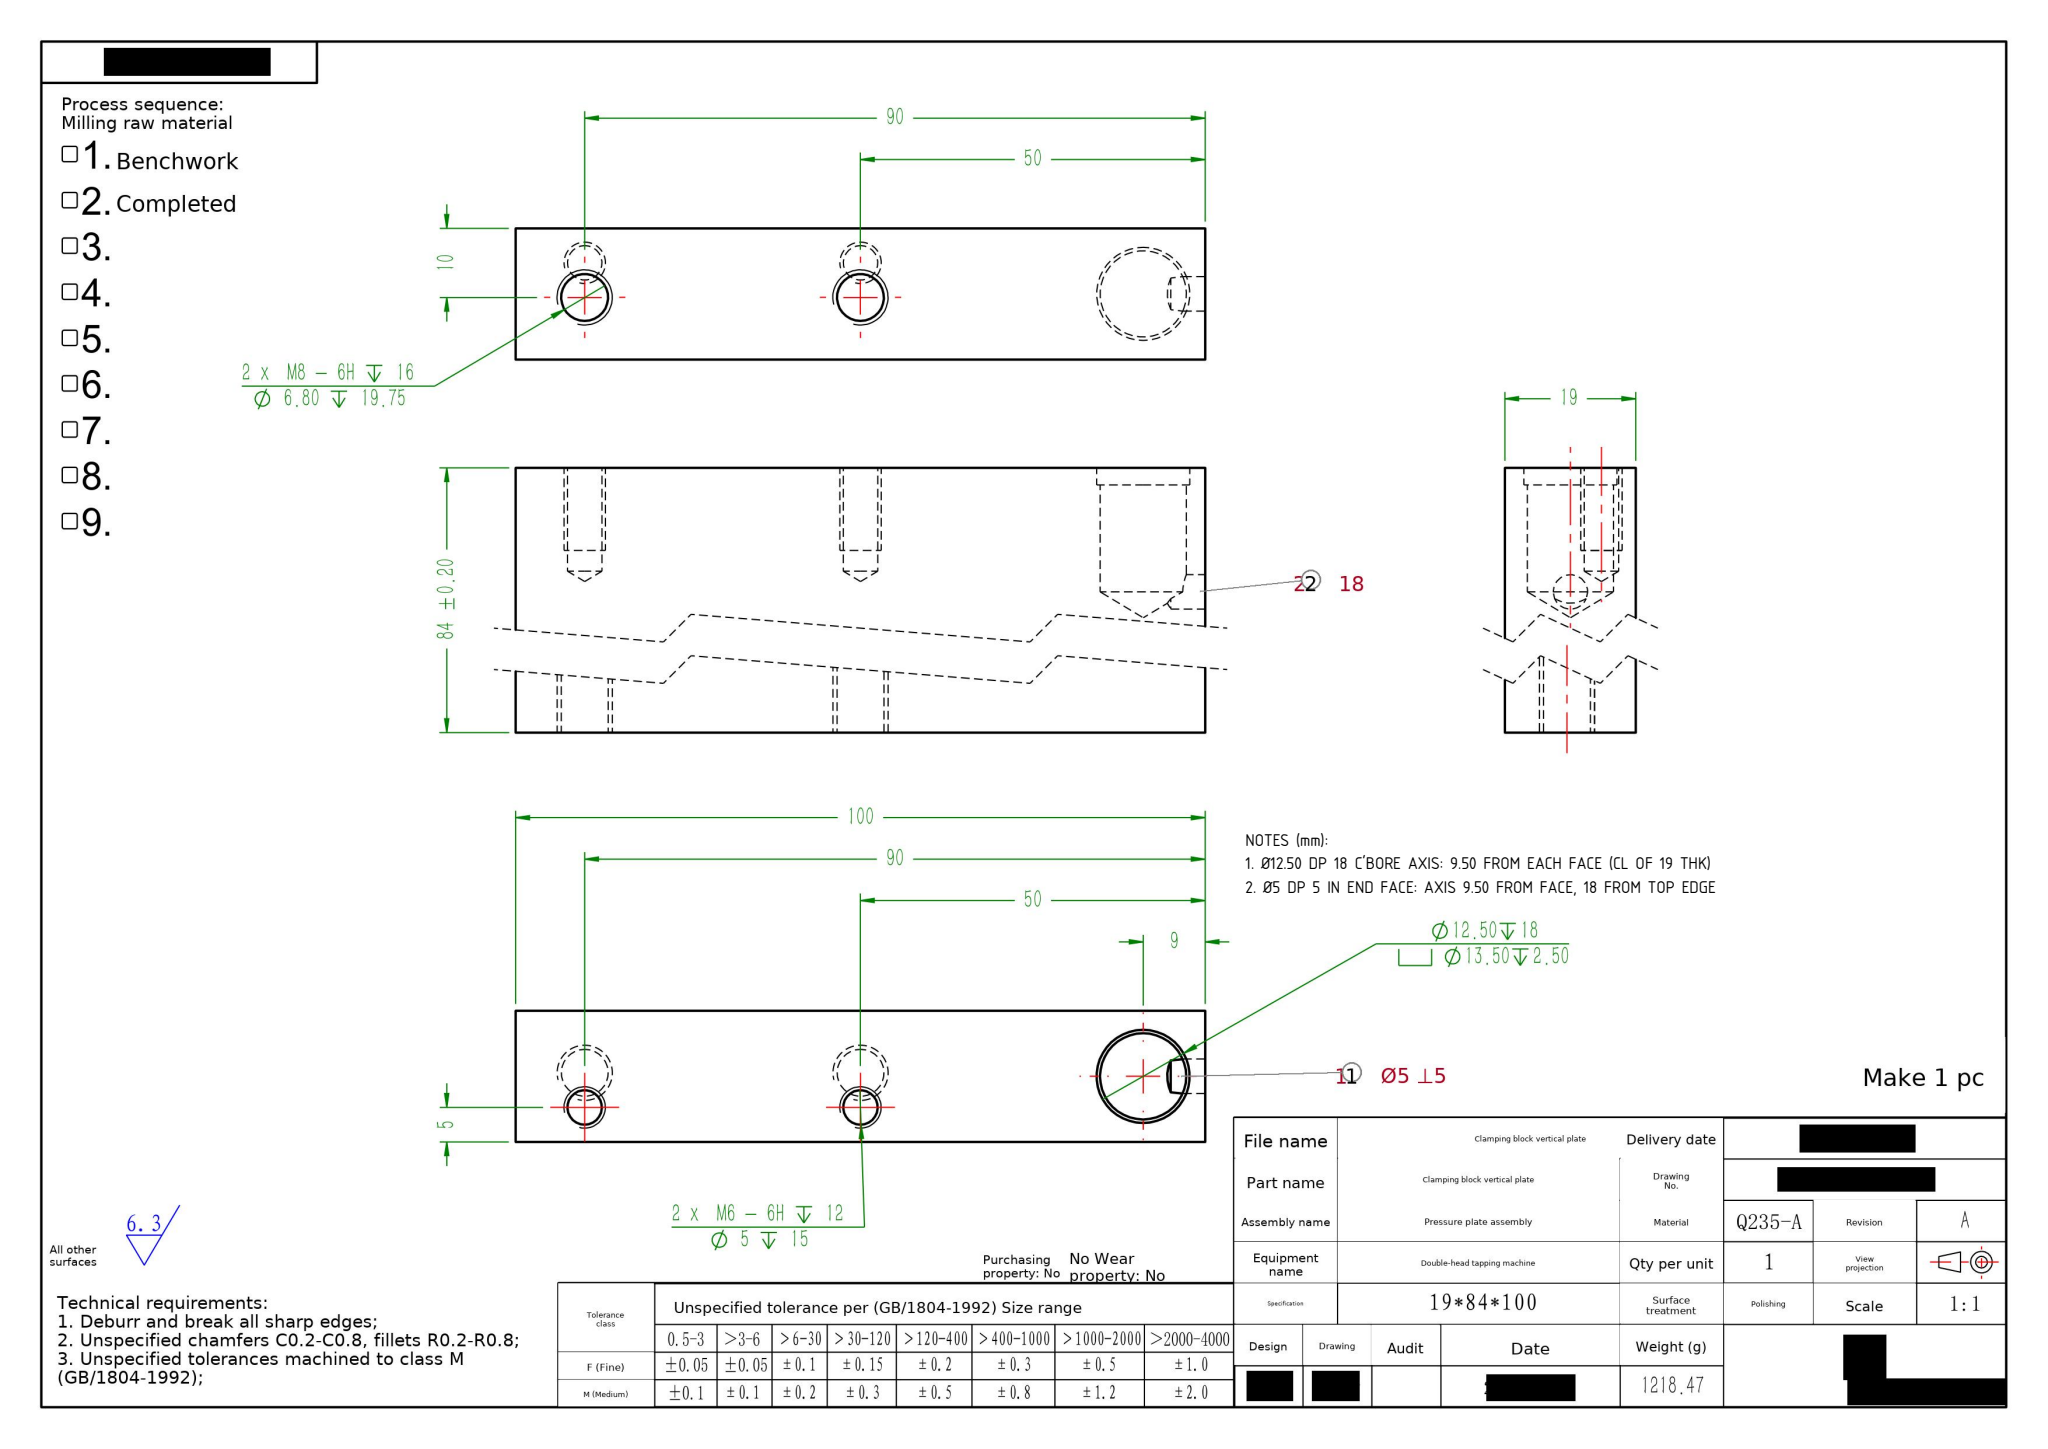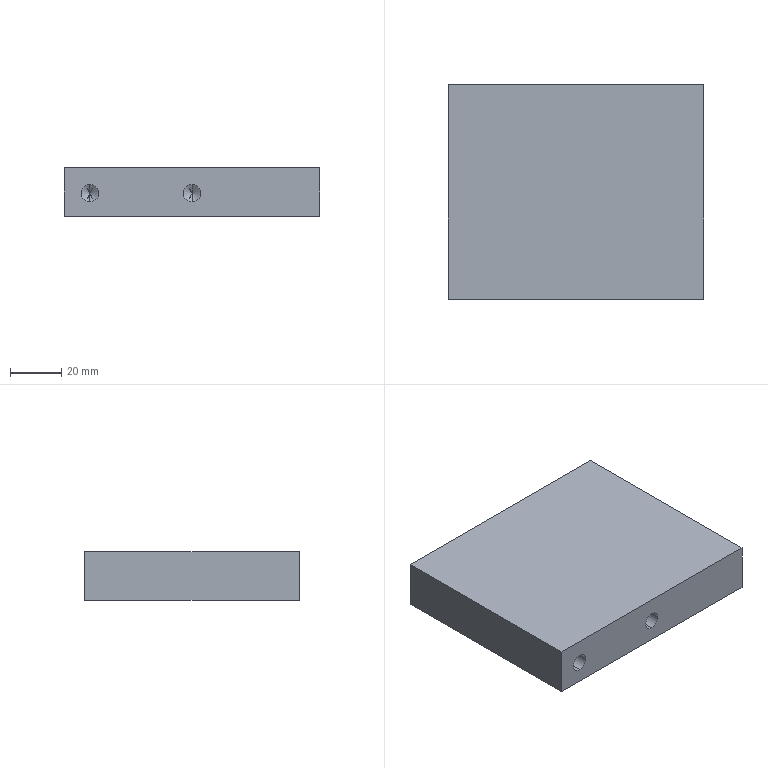Part | SolidWorks | mm | material Q235-A | 1 solid | 32 faces | box 100 x 84 x 19 mm | volume 155022 mm3 | cylinder 14 | cone 11 | plane 7 | commonest cylinder face diameters 5 x6 6.8 x4 13.5 x2 12.5 x2
Drawing notes:
Ø12.50 DP 18 C'BORE AXIS: 9.50 FROM EACH FACE (CL OF 19 THK) | from the solid: cyl Ø12.5 & Ø13.5, axis y, pos [x=91, z=9.5]; bbox z=19 -> 9.5 both faces
Ø5 DP 5 IN END FACE: AXIS 9.50 FROM FACE, 18 FROM TOP EDGE | from the solid: cyl Ø5 axis x at [y=66, z=9.5], L=5 from x=100 end face; bbox y=84 -> 84-66=18; z 9.5 of 19
build123d program:
from build123d import *

# Parameters (mm, degrees)
SKETCH1_W                         = 100
SKETCH1_H                         = 19
BOSS_EXTRUDE1_DEPTH               = 84
HOLE1_D                           = 12.5
HOLE1_DEPTH                       = 18
HOLE1_CBORE_D                     = 13.5
HOLE1_CBORE_DEPTH                 = 2.5
HOLE1_TIP                         = 3.755
M8_TAPPED_HOLE2_D                 = 6.8
M8_TAPPED_HOLE2_DEPTH             = 19.75
M8_TAPPED_HOLE2_TIP               = 2.043
M6_TAPPED_HOLE1_D                 = 5
M6_TAPPED_HOLE1_DEPTH             = 15
M6_TAPPED_HOLE1_TIP               = 1.502
M6_THREADED_HOLE_DRILL_BIT1_D     = 5
M6_THREADED_HOLE_DRILL_BIT1_DEPTH = 5
M6_THREADED_HOLE_DRILL_BIT1_TIP   = 1.502


with BuildPart() as part:
    # Sketch1 → Boss-Extrude1 (new body)
    with BuildSketch(Plane(origin=(0, 0, 0), x_dir=(1, 0, 0), z_dir=(0, 1, 0))):
        Rectangle(SKETCH1_W, SKETCH1_H)
    extrude(amount=BOSS_EXTRUDE1_DEPTH)

    # Hole1
    with Locations(Plane(origin=(0, 84, 0), x_dir=(1, 0, 0), z_dir=(0, 1, 0))):
        with Locations((41, 0)):
            CounterBoreHole(HOLE1_D / 2, HOLE1_CBORE_D / 2, HOLE1_CBORE_DEPTH, depth=HOLE1_DEPTH)
            with Locations((0, 0, -(HOLE1_DEPTH + HOLE1_TIP / 2))):  # 118° drill point
                Cone(0, HOLE1_D / 2, HOLE1_TIP, mode=Mode.SUBTRACT)

    # M8 Tapped Hole2
    with Locations(Plane(origin=(0, 0, 0), x_dir=(-1, 0, 0), z_dir=(0, -1, 0))):
        with Locations((40, 0.5), (0, 0.5)):
            Hole(M8_TAPPED_HOLE2_D / 2, depth=M8_TAPPED_HOLE2_DEPTH)
            with Locations((0, 0, -(M8_TAPPED_HOLE2_DEPTH + M8_TAPPED_HOLE2_TIP / 2))):  # 118° drill point
                Cone(0, M8_TAPPED_HOLE2_D / 2, M8_TAPPED_HOLE2_TIP, mode=Mode.SUBTRACT)

    # M6 Tapped Hole1
    with Locations(Plane(origin=(0, 84, 0), x_dir=(1, 0, 0), z_dir=(0, 1, 0))):
        with Locations((-40, -4.5), (0, -4.5)):
            Hole(M6_TAPPED_HOLE1_D / 2, depth=M6_TAPPED_HOLE1_DEPTH)
            with Locations((0, 0, -(M6_TAPPED_HOLE1_DEPTH + M6_TAPPED_HOLE1_TIP / 2))):  # 118° drill point
                Cone(0, M6_TAPPED_HOLE1_D / 2, M6_TAPPED_HOLE1_TIP, mode=Mode.SUBTRACT)

    # M6 Threaded Hole Drill Bit1
    with Locations(Plane(origin=(50, 0, 0), x_dir=(0, 0, -1), z_dir=(1, 0, 0))):
        with Locations((0, 66)):
            Hole(M6_THREADED_HOLE_DRILL_BIT1_D / 2, depth=M6_THREADED_HOLE_DRILL_BIT1_DEPTH)
            with Locations((0, 0, -(M6_THREADED_HOLE_DRILL_BIT1_DEPTH + M6_THREADED_HOLE_DRILL_BIT1_TIP / 2))):  # 118° drill point
                Cone(0, M6_THREADED_HOLE_DRILL_BIT1_D / 2, M6_THREADED_HOLE_DRILL_BIT1_TIP, mode=Mode.SUBTRACT)


solid = part.part
STEP:
#1=CARTESIAN_POINT('',(46.728,66.,2.5));
#2=VERTEX_POINT('',#1);
#3=CARTESIAN_POINT('',(45.,65.017,2.298));
#4=VERTEX_POINT('',#3);
#5=CARTESIAN_POINT('',(46.728,66.,2.5));
#6=CARTESIAN_POINT('',(46.435,65.839,2.5));
#7=CARTESIAN_POINT('',(46.144,65.677,2.485));
#8=CARTESIAN_POINT('',(45.567,65.35,2.42));
#9=CARTESIAN_POINT('',(45.282,65.185,2.37));
#10=CARTESIAN_POINT('',(45.,65.017,2.298));
#11=B_SPLINE_CURVE_WITH_KNOTS('',3,(#5,#6,#7,#8,#9,#10),.UNSPECIFIED.,.F.,.F.,(4,2,4),(0.0005174,0.001517,0.002516),.UNSPECIFIED.);
#12=EDGE_CURVE('',#2,#4,#11,.T.);
#13=ORIENTED_EDGE('',*,*,#12,.F.);
#14=CARTESIAN_POINT('',(50.,66.,2.5));
#15=VERTEX_POINT('',#14);
#16=CARTESIAN_POINT('',(50.,66.,2.5));
#17=DIRECTION('',(1.,0.,0.));
#18=VECTOR('',#17,1000.);
#19=LINE('',#16,#18);
#20=EDGE_CURVE('',#2,#15,#19,.T.);
#21=ORIENTED_EDGE('',*,*,#20,.T.);
#22=CARTESIAN_POINT('',(50.,66.,-2.5));
#23=VERTEX_POINT('',#22);
#24=CARTESIAN_POINT('',(50.,66.,0.));
#25=DIRECTION('',(1.,0.,0.));
#26=DIRECTION('',(0.,0.,-1.));
#27=AXIS2_PLACEMENT_3D('',#24,#25,#26);
#28=CIRCLE('',#27,2.5);
#29=EDGE_CURVE('',#15,#23,#28,.T.);
#30=ORIENTED_EDGE('',*,*,#29,.T.);
#31=CARTESIAN_POINT('',(46.728,66.,-2.5));
#32=VERTEX_POINT('',#31);
#33=CARTESIAN_POINT('',(50.,66.,-2.5));
#34=DIRECTION('',(1.,0.,0.));
#35=VECTOR('',#34,1000.);
#36=LINE('',#33,#35);
#37=EDGE_CURVE('',#32,#23,#36,.T.);
#38=ORIENTED_EDGE('',*,*,#37,.F.);
#39=CARTESIAN_POINT('',(45.,65.017,-2.298));
#40=VERTEX_POINT('',#39);
#41=CARTESIAN_POINT('',(45.,65.017,-2.298));
#42=CARTESIAN_POINT('',(45.282,65.185,-2.37));
#43=CARTESIAN_POINT('',(45.567,65.35,-2.42));
#44=CARTESIAN_POINT('',(46.144,65.677,-2.485));
#45=CARTESIAN_POINT('',(46.435,65.839,-2.5));
#46=CARTESIAN_POINT('',(46.728,66.,-2.5));
#47=B_SPLINE_CURVE_WITH_KNOTS('',3,(#41,#42,#43,#44,#45,#46),.UNSPECIFIED.,.F.,.F.,(4,2,4),(0.0002676,0.001267,0.002266),.UNSPECIFIED.);
#48=EDGE_CURVE('',#40,#32,#47,.T.);
#49=ORIENTED_EDGE('',*,*,#48,.F.);
#50=CARTESIAN_POINT('',(45.,66.,0.));
#51=DIRECTION('',(1.,0.,0.));
#52=DIRECTION('',(0.,0.,-1.));
#53=AXIS2_PLACEMENT_3D('',#50,#51,#52);
#54=CIRCLE('',#53,2.5);
#55=EDGE_CURVE('',#4,#40,#54,.T.);
#56=ORIENTED_EDGE('',*,*,#55,.F.);
#57=EDGE_LOOP('',(#13,#21,#30,#38,#49,#56));
#58=FACE_OUTER_BOUND('',#57,.T.);
#59=CARTESIAN_POINT('',(50.,66.,0.));
#60=DIRECTION('',(1.,0.,0.));
#61=DIRECTION('',(0.,0.,-1.));
#62=AXIS2_PLACEMENT_3D('',#59,#60,#61);
#63=CYLINDRICAL_SURFACE('',#62,2.5);
#64=ADVANCED_FACE('',(#58),#63,.F.);
#65=CARTESIAN_POINT('',(-40.,69.,2.));
#66=VERTEX_POINT('',#65);
#67=CARTESIAN_POINT('',(-40.,69.,7.));
#68=VERTEX_POINT('',#67);
#69=CARTESIAN_POINT('',(-40.,69.,4.5));
#70=DIRECTION('',(0.,1.,0.));
#71=DIRECTION('',(0.,0.,1.));
#72=AXIS2_PLACEMENT_3D('',#69,#70,#71);
#73=CIRCLE('',#72,2.5);
#74=EDGE_CURVE('',#66,#68,#73,.T.);
#75=ORIENTED_EDGE('',*,*,#74,.F.);
#76=CARTESIAN_POINT('',(-40.,84.,2.));
#77=VERTEX_POINT('',#76);
#78=CARTESIAN_POINT('',(-40.,84.,2.));
#79=DIRECTION('',(0.,1.,0.));
#80=VECTOR('',#79,1000.);
#81=LINE('',#78,#80);
#82=EDGE_CURVE('',#66,#77,#81,.T.);
#83=ORIENTED_EDGE('',*,*,#82,.T.);
#84=CARTESIAN_POINT('',(-40.,84.,7.));
#85=VERTEX_POINT('',#84);
#86=CARTESIAN_POINT('',(-40.,84.,4.5));
#87=DIRECTION('',(0.,1.,0.));
#88=DIRECTION('',(0.,0.,1.));
#89=AXIS2_PLACEMENT_3D('',#86,#87,#88);
#90=CIRCLE('',#89,2.5);
#91=EDGE_CURVE('',#77,#85,#90,.T.);
#92=ORIENTED_EDGE('',*,*,#91,.T.);
#93=CARTESIAN_POINT('',(-40.,84.,7.));
#94=DIRECTION('',(0.,1.,0.));
#95=VECTOR('',#94,1000.);
#96=LINE('',#93,#95);
#97=EDGE_CURVE('',#68,#85,#96,.T.);
#98=ORIENTED_EDGE('',*,*,#97,.F.);
#99=EDGE_LOOP('',(#75,#83,#92,#98));
#100=FACE_OUTER_BOUND('',#99,.T.);
#101=CARTESIAN_POINT('',(-40.,84.,4.5));
#102=DIRECTION('',(0.,1.,0.));
#103=DIRECTION('',(0.,0.,1.));
#104=AXIS2_PLACEMENT_3D('',#101,#102,#103);
#105=CYLINDRICAL_SURFACE('',#104,2.5);
#106=ADVANCED_FACE('',(#100),#105,.F.);
#107=CARTESIAN_POINT('',(-40.,67.498,4.5));
#108=VERTEX_POINT('',#107);
#109=CARTESIAN_POINT('',(-40.,69.,7.));
#110=DIRECTION('',(0.,0.515,0.8572));
#111=VECTOR('',#110,1000.);
#112=LINE('',#109,#111);
#113=EDGE_CURVE('',#108,#68,#112,.T.);
#114=ORIENTED_EDGE('',*,*,#113,.F.);
#115=CARTESIAN_POINT('',(-40.,69.,2.));
#116=DIRECTION('',(0.,0.515,-0.8572));
#117=VECTOR('',#116,1000.);
#118=LINE('',#115,#117);
#119=EDGE_CURVE('',#108,#66,#118,.T.);
#120=ORIENTED_EDGE('',*,*,#119,.T.);
#121=ORIENTED_EDGE('',*,*,#74,.T.);
#122=EDGE_LOOP('',(#114,#120,#121));
#123=FACE_OUTER_BOUND('',#122,.T.);
#124=CARTESIAN_POINT('',(-40.,69.,4.5));
#125=DIRECTION('',(0.,1.,0.));
#126=DIRECTION('',(0.,0.,1.));
#127=AXIS2_PLACEMENT_3D('',#124,#125,#126);
#128=CONICAL_SURFACE('',#127,2.5,1.03);
#129=ADVANCED_FACE('',(#123),#128,.F.);
#130=CARTESIAN_POINT('',(0.,69.,2.));
#131=VERTEX_POINT('',#130);
#132=CARTESIAN_POINT('',(0.,69.,7.));
#133=VERTEX_POINT('',#132);
#134=CARTESIAN_POINT('',(0.,69.,4.5));
#135=DIRECTION('',(0.,1.,0.));
#136=DIRECTION('',(0.,0.,1.));
#137=AXIS2_PLACEMENT_3D('',#134,#135,#136);
#138=CIRCLE('',#137,2.5);
#139=EDGE_CURVE('',#131,#133,#138,.T.);
#140=ORIENTED_EDGE('',*,*,#139,.F.);
#141=CARTESIAN_POINT('',(0.,84.,2.));
#142=VERTEX_POINT('',#141);
#143=CARTESIAN_POINT('',(0.,84.,2.));
#144=DIRECTION('',(0.,1.,0.));
#145=VECTOR('',#144,1000.);
#146=LINE('',#143,#145);
#147=EDGE_CURVE('',#131,#142,#146,.T.);
#148=ORIENTED_EDGE('',*,*,#147,.T.);
#149=CARTESIAN_POINT('',(0.,84.,7.));
#150=VERTEX_POINT('',#149);
#151=CARTESIAN_POINT('',(0.,84.,4.5));
#152=DIRECTION('',(0.,1.,0.));
#153=DIRECTION('',(0.,0.,1.));
#154=AXIS2_PLACEMENT_3D('',#151,#152,#153);
#155=CIRCLE('',#154,2.5);
#156=EDGE_CURVE('',#142,#150,#155,.T.);
#157=ORIENTED_EDGE('',*,*,#156,.T.);
#158=CARTESIAN_POINT('',(0.,84.,7.));
#159=DIRECTION('',(0.,1.,0.));
#160=VECTOR('',#159,1000.);
#161=LINE('',#158,#160);
#162=EDGE_CURVE('',#133,#150,#161,.T.);
#163=ORIENTED_EDGE('',*,*,#162,.F.);
#164=EDGE_LOOP('',(#140,#148,#157,#163));
#165=FACE_OUTER_BOUND('',#164,.T.);
#166=CARTESIAN_POINT('',(0.,84.,4.5));
#167=DIRECTION('',(0.,1.,0.));
#168=DIRECTION('',(0.,0.,1.));
#169=AXIS2_PLACEMENT_3D('',#166,#167,#168);
#170=CYLINDRICAL_SURFACE('',#169,2.5);
#171=ADVANCED_FACE('',(#165),#170,.F.);
#172=CARTESIAN_POINT('',(0.,67.498,4.5));
#173=VERTEX_POINT('',#172);
#174=CARTESIAN_POINT('',(0.,69.,7.));
#175=DIRECTION('',(0.,0.515,0.8572));
#176=VECTOR('',#175,1000.);
#177=LINE('',#174,#176);
#178=EDGE_CURVE('',#173,#133,#177,.T.);
#179=ORIENTED_EDGE('',*,*,#178,.F.);
#180=CARTESIAN_POINT('',(0.,69.,2.));
#181=DIRECTION('',(0.,0.515,-0.8572));
#182=VECTOR('',#181,1000.);
#183=LINE('',#180,#182);
#184=EDGE_CURVE('',#173,#131,#183,.T.);
#185=ORIENTED_EDGE('',*,*,#184,.T.);
#186=ORIENTED_EDGE('',*,*,#139,.T.);
#187=EDGE_LOOP('',(#179,#185,#186));
#188=FACE_OUTER_BOUND('',#187,.T.);
#189=CARTESIAN_POINT('',(0.,69.,4.5));
#190=DIRECTION('',(0.,1.,0.));
#191=DIRECTION('',(0.,0.,1.));
#192=AXIS2_PLACEMENT_3D('',#189,#190,#191);
#193=CONICAL_SURFACE('',#192,2.5,1.03);
#194=ADVANCED_FACE('',(#188),#193,.F.);
#195=CARTESIAN_POINT('',(0.,19.75,2.9));
#196=VERTEX_POINT('',#195);
#197=CARTESIAN_POINT('',(0.,19.75,-3.9));
#198=VERTEX_POINT('',#197);
#199=CARTESIAN_POINT('',(0.,19.75,-0.5));
#200=DIRECTION('',(0.,-1.,0.));
#201=DIRECTION('',(0.,0.,-1.));
#202=AXIS2_PLACEMENT_3D('',#199,#200,#201);
#203=CIRCLE('',#202,3.4);
#204=EDGE_CURVE('',#196,#198,#203,.T.);
#205=ORIENTED_EDGE('',*,*,#204,.F.);
#206=CARTESIAN_POINT('',(0.,-0.,2.9));
#207=VERTEX_POINT('',#206);
#208=CARTESIAN_POINT('',(0.,0.,2.9));
#209=DIRECTION('',(0.,-1.,0.));
#210=VECTOR('',#209,1000.);
#211=LINE('',#208,#210);
#212=EDGE_CURVE('',#196,#207,#211,.T.);
#213=ORIENTED_EDGE('',*,*,#212,.T.);
#214=CARTESIAN_POINT('',(0.,-0.,-3.9));
#215=VERTEX_POINT('',#214);
#216=CARTESIAN_POINT('',(0.,-0.,-0.5));
#217=DIRECTION('',(0.,-1.,0.));
#218=DIRECTION('',(0.,0.,-1.));
#219=AXIS2_PLACEMENT_3D('',#216,#217,#218);
#220=CIRCLE('',#219,3.4);
#221=EDGE_CURVE('',#207,#215,#220,.T.);
#222=ORIENTED_EDGE('',*,*,#221,.T.);
#223=CARTESIAN_POINT('',(0.,0.,-3.9));
#224=DIRECTION('',(0.,-1.,0.));
#225=VECTOR('',#224,1000.);
#226=LINE('',#223,#225);
#227=EDGE_CURVE('',#198,#215,#226,.T.);
#228=ORIENTED_EDGE('',*,*,#227,.F.);
#229=EDGE_LOOP('',(#205,#213,#222,#228));
#230=FACE_OUTER_BOUND('',#229,.T.);
#231=CARTESIAN_POINT('',(0.,0.,-0.5));
#232=DIRECTION('',(0.,-1.,0.));
#233=DIRECTION('',(0.,0.,-1.));
#234=AXIS2_PLACEMENT_3D('',#231,#232,#233);
#235=CYLINDRICAL_SURFACE('',#234,3.4);
#236=ADVANCED_FACE('',(#230),#235,.F.);
#237=CARTESIAN_POINT('',(-0.,21.793,-0.5));
#238=VERTEX_POINT('',#237);
#239=CARTESIAN_POINT('',(0.,19.75,-3.9));
#240=DIRECTION('',(0.,-0.515,-0.8572));
#241=VECTOR('',#240,1000.);
#242=LINE('',#239,#241);
#243=EDGE_CURVE('',#238,#198,#242,.T.);
#244=ORIENTED_EDGE('',*,*,#243,.F.);
#245=CARTESIAN_POINT('',(0.,19.75,2.9));
#246=DIRECTION('',(0.,-0.515,0.8572));
#247=VECTOR('',#246,1000.);
#248=LINE('',#245,#247);
#249=EDGE_CURVE('',#238,#196,#248,.T.);
#250=ORIENTED_EDGE('',*,*,#249,.T.);
#251=ORIENTED_EDGE('',*,*,#204,.T.);
#252=EDGE_LOOP('',(#244,#250,#251));
#253=FACE_OUTER_BOUND('',#252,.T.);
#254=CARTESIAN_POINT('',(0.,19.75,-0.5));
#255=DIRECTION('',(0.,-1.,0.));
#256=DIRECTION('',(0.,0.,-1.));
#257=AXIS2_PLACEMENT_3D('',#254,#255,#256);
#258=CONICAL_SURFACE('',#257,3.4,1.03);
#259=ADVANCED_FACE('',(#253),#258,.F.);
#260=CARTESIAN_POINT('',(-40.,19.75,2.9));
#261=VERTEX_POINT('',#260);
#262=CARTESIAN_POINT('',(-40.,19.75,-3.9));
#263=VERTEX_POINT('',#262);
#264=CARTESIAN_POINT('',(-40.,19.75,-0.5));
#265=DIRECTION('',(0.,-1.,0.));
#266=DIRECTION('',(0.,0.,-1.));
#267=AXIS2_PLACEMENT_3D('',#264,#265,#266);
#268=CIRCLE('',#267,3.4);
#269=EDGE_CURVE('',#261,#263,#268,.T.);
#270=ORIENTED_EDGE('',*,*,#269,.F.);
#271=CARTESIAN_POINT('',(-40.,-0.,2.9));
#272=VERTEX_POINT('',#271);
#273=CARTESIAN_POINT('',(-40.,0.,2.9));
#274=DIRECTION('',(0.,-1.,0.));
#275=VECTOR('',#274,1000.);
#276=LINE('',#273,#275);
#277=EDGE_CURVE('',#261,#272,#276,.T.);
#278=ORIENTED_EDGE('',*,*,#277,.T.);
#279=CARTESIAN_POINT('',(-40.,-0.,-3.9));
#280=VERTEX_POINT('',#279);
#281=CARTESIAN_POINT('',(-40.,-0.,-0.5));
#282=DIRECTION('',(0.,-1.,0.));
#283=DIRECTION('',(0.,0.,-1.));
#284=AXIS2_PLACEMENT_3D('',#281,#282,#283);
#285=CIRCLE('',#284,3.4);
#286=EDGE_CURVE('',#272,#280,#285,.T.);
#287=ORIENTED_EDGE('',*,*,#286,.T.);
#288=CARTESIAN_POINT('',(-40.,0.,-3.9));
#289=DIRECTION('',(0.,-1.,0.));
#290=VECTOR('',#289,1000.);
#291=LINE('',#288,#290);
#292=EDGE_CURVE('',#263,#280,#291,.T.);
#293=ORIENTED_EDGE('',*,*,#292,.F.);
#294=EDGE_LOOP('',(#270,#278,#287,#293));
#295=FACE_OUTER_BOUND('',#294,.T.);
#296=CARTESIAN_POINT('',(-40.,0.,-0.5));
#297=DIRECTION('',(0.,-1.,0.));
#298=DIRECTION('',(0.,0.,-1.));
#299=AXIS2_PLACEMENT_3D('',#296,#297,#298);
#300=CYLINDRICAL_SURFACE('',#299,3.4);
#301=ADVANCED_FACE('',(#295),#300,.F.);
#302=CARTESIAN_POINT('',(-40.,21.793,-0.5));
#303=VERTEX_POINT('',#302);
#304=CARTESIAN_POINT('',(-40.,19.75,-3.9));
#305=DIRECTION('',(0.,-0.515,-0.8572));
#306=VECTOR('',#305,1000.);
#307=LINE('',#304,#306);
#308=EDGE_CURVE('',#303,#263,#307,.T.);
#309=ORIENTED_EDGE('',*,*,#308,.F.);
#310=CARTESIAN_POINT('',(-40.,19.75,2.9));
#311=DIRECTION('',(0.,-0.515,0.8572));
#312=VECTOR('',#311,1000.);
#313=LINE('',#310,#312);
#314=EDGE_CURVE('',#303,#261,#313,.T.);
#315=ORIENTED_EDGE('',*,*,#314,.T.);
#316=ORIENTED_EDGE('',*,*,#269,.T.);
#317=EDGE_LOOP('',(#309,#315,#316));
#318=FACE_OUTER_BOUND('',#317,.T.);
#319=CARTESIAN_POINT('',(-40.,19.75,-0.5));
#320=DIRECTION('',(0.,-1.,0.));
#321=DIRECTION('',(0.,0.,-1.));
#322=AXIS2_PLACEMENT_3D('',#319,#320,#321);
#323=CONICAL_SURFACE('',#322,3.4,1.03);
#324=ADVANCED_FACE('',(#318),#323,.F.);
#325=CARTESIAN_POINT('',(41.,81.5,-6.75));
#326=VERTEX_POINT('',#325);
#327=CARTESIAN_POINT('',(41.,81.5,6.75));
#328=VERTEX_POINT('',#327);
#329=CARTESIAN_POINT('',(41.,81.5,0.));
#330=DIRECTION('',(0.,1.,0.));
#331=DIRECTION('',(0.,0.,1.));
#332=AXIS2_PLACEMENT_3D('',#329,#330,#331);
#333=CIRCLE('',#332,6.75);
#334=EDGE_CURVE('',#326,#328,#333,.T.);
#335=ORIENTED_EDGE('',*,*,#334,.F.);
#336=CARTESIAN_POINT('',(41.,84.,-6.75));
#337=VERTEX_POINT('',#336);
#338=CARTESIAN_POINT('',(41.,84.,-6.75));
#339=DIRECTION('',(0.,1.,0.));
#340=VECTOR('',#339,1000.);
#341=LINE('',#338,#340);
#342=EDGE_CURVE('',#326,#337,#341,.T.);
#343=ORIENTED_EDGE('',*,*,#342,.T.);
#344=CARTESIAN_POINT('',(41.,84.,6.75));
#345=VERTEX_POINT('',#344);
#346=CARTESIAN_POINT('',(41.,84.,0.));
#347=DIRECTION('',(0.,1.,0.));
#348=DIRECTION('',(0.,0.,1.));
#349=AXIS2_PLACEMENT_3D('',#346,#347,#348);
#350=CIRCLE('',#349,6.75);
#351=EDGE_CURVE('',#337,#345,#350,.T.);
#352=ORIENTED_EDGE('',*,*,#351,.T.);
#353=CARTESIAN_POINT('',(41.,84.,6.75));
#354=DIRECTION('',(0.,1.,0.));
#355=VECTOR('',#354,1000.);
#356=LINE('',#353,#355);
#357=EDGE_CURVE('',#328,#345,#356,.T.);
#358=ORIENTED_EDGE('',*,*,#357,.F.);
#359=EDGE_LOOP('',(#335,#343,#352,#358));
#360=FACE_OUTER_BOUND('',#359,.T.);
#361=CARTESIAN_POINT('',(41.,84.,0.));
#362=DIRECTION('',(0.,1.,0.));
#363=DIRECTION('',(0.,0.,1.));
#364=AXIS2_PLACEMENT_3D('',#361,#362,#363);
#365=CYLINDRICAL_SURFACE('',#364,6.75);
#366=ADVANCED_FACE('',(#360),#365,.F.);
#367=CARTESIAN_POINT('',(41.,66.,-6.25));
#368=VERTEX_POINT('',#367);
#369=CARTESIAN_POINT('',(41.,66.,6.25));
#370=VERTEX_POINT('',#369);
#371=CARTESIAN_POINT('',(41.,66.,0.));
#372=DIRECTION('',(0.,1.,0.));
#373=DIRECTION('',(0.,0.,1.));
#374=AXIS2_PLACEMENT_3D('',#371,#372,#373);
#375=CIRCLE('',#374,6.25);
#376=EDGE_CURVE('',#368,#370,#375,.T.);
#377=ORIENTED_EDGE('',*,*,#376,.F.);
#378=CARTESIAN_POINT('',(41.,81.5,-6.25));
#379=VERTEX_POINT('',#378);
#380=CARTESIAN_POINT('',(41.,84.,-6.25));
#381=DIRECTION('',(0.,1.,0.));
#382=VECTOR('',#381,1000.);
#383=LINE('',#380,#382);
#384=EDGE_CURVE('',#368,#379,#383,.T.);
#385=ORIENTED_EDGE('',*,*,#384,.T.);
#386=CARTESIAN_POINT('',(41.,81.5,6.25));
#387=VERTEX_POINT('',#386);
#388=CARTESIAN_POINT('',(41.,81.5,0.));
#389=DIRECTION('',(0.,1.,0.));
#390=DIRECTION('',(0.,0.,1.));
#391=AXIS2_PLACEMENT_3D('',#388,#389,#390);
#392=CIRCLE('',#391,6.25);
#393=EDGE_CURVE('',#379,#387,#392,.T.);
#394=ORIENTED_EDGE('',*,*,#393,.T.);
#395=CARTESIAN_POINT('',(41.,84.,6.25));
#396=DIRECTION('',(0.,1.,0.));
#397=VECTOR('',#396,1000.);
#398=LINE('',#395,#397);
#399=EDGE_CURVE('',#370,#387,#398,.T.);
#400=ORIENTED_EDGE('',*,*,#399,.F.);
#401=EDGE_LOOP('',(#377,#385,#394,#400));
#402=FACE_OUTER_BOUND('',#401,.T.);
#403=CARTESIAN_POINT('',(41.,84.,0.));
#404=DIRECTION('',(0.,1.,0.));
#405=DIRECTION('',(0.,0.,1.));
#406=AXIS2_PLACEMENT_3D('',#403,#404,#405);
#407=CYLINDRICAL_SURFACE('',#406,6.25);
#408=ADVANCED_FACE('',(#402),#407,.F.);
#409=CARTESIAN_POINT('',(41.,62.245,0.));
#410=VERTEX_POINT('',#409);
#411=CARTESIAN_POINT('',(41.,66.,6.25));
#412=DIRECTION('',(0.,0.515,0.8572));
#413=VECTOR('',#412,1000.);
#414=LINE('',#411,#413);
#415=EDGE_CURVE('',#410,#370,#414,.T.);
#416=ORIENTED_EDGE('',*,*,#415,.F.);
#417=CARTESIAN_POINT('',(41.,66.,-6.25));
#418=DIRECTION('',(0.,0.515,-0.8572));
#419=VECTOR('',#418,1000.);
#420=LINE('',#417,#419);
#421=EDGE_CURVE('',#410,#368,#420,.T.);
#422=ORIENTED_EDGE('',*,*,#421,.T.);
#423=ORIENTED_EDGE('',*,*,#376,.T.);
#424=EDGE_LOOP('',(#416,#422,#423));
#425=FACE_OUTER_BOUND('',#424,.T.);
#426=CARTESIAN_POINT('',(41.,66.,0.));
#427=DIRECTION('',(0.,1.,0.));
#428=DIRECTION('',(0.,0.,1.));
#429=AXIS2_PLACEMENT_3D('',#426,#427,#428);
#430=CONICAL_SURFACE('',#429,6.25,1.03);
#431=ADVANCED_FACE('',(#425),#430,.F.);
#432=CARTESIAN_POINT('',(-50.,0.,-9.5));
#433=VERTEX_POINT('',#432);
#434=CARTESIAN_POINT('',(-50.,0.,9.5));
#435=VERTEX_POINT('',#434);
#436=CARTESIAN_POINT('',(-50.,0.,-9.5));
#437=DIRECTION('',(0.,0.,1.));
#438=VECTOR('',#437,1000.);
#439=LINE('',#436,#438);
#440=EDGE_CURVE('',#433,#435,#439,.T.);
#441=ORIENTED_EDGE('',*,*,#440,.T.);
#442=CARTESIAN_POINT('',(-50.,84.,9.5));
#443=VERTEX_POINT('',#442);
#444=CARTESIAN_POINT('',(-50.,84.,9.5));
#445=DIRECTION('',(0.,-1.,0.));
#446=VECTOR('',#445,1000.);
#447=LINE('',#444,#446);
#448=EDGE_CURVE('',#443,#435,#447,.T.);
#449=ORIENTED_EDGE('',*,*,#448,.F.);
#450=CARTESIAN_POINT('',(-50.,84.,-9.5));
#451=VERTEX_POINT('',#450);
#452=CARTESIAN_POINT('',(-50.,84.,-9.5));
#453=DIRECTION('',(0.,0.,1.));
#454=VECTOR('',#453,1000.);
#455=LINE('',#452,#454);
#456=EDGE_CURVE('',#451,#443,#455,.T.);
#457=ORIENTED_EDGE('',*,*,#456,.F.);
#458=CARTESIAN_POINT('',(-50.,84.,-9.5));
#459=DIRECTION('',(0.,-1.,0.));
#460=VECTOR('',#459,1000.);
#461=LINE('',#458,#460);
#462=EDGE_CURVE('',#451,#433,#461,.T.);
#463=ORIENTED_EDGE('',*,*,#462,.T.);
#464=EDGE_LOOP('',(#441,#449,#457,#463));
#465=FACE_OUTER_BOUND('',#464,.T.);
#466=CARTESIAN_POINT('',(-50.,84.,-9.5));
#467=DIRECTION('',(1.,0.,0.));
#468=DIRECTION('',(0.,0.,-1.));
#469=AXIS2_PLACEMENT_3D('',#466,#467,#468);
#470=PLANE('',#469);
#471=ADVANCED_FACE('',(#465),#470,.F.);
#472=CARTESIAN_POINT('',(50.,0.,9.5));
#473=VERTEX_POINT('',#472);
#474=CARTESIAN_POINT('',(50.,0.,9.5));
#475=DIRECTION('',(1.,0.,0.));
#476=VECTOR('',#475,1000.);
#477=LINE('',#474,#476);
#478=EDGE_CURVE('',#435,#473,#477,.T.);
#479=ORIENTED_EDGE('',*,*,#478,.T.);
#480=CARTESIAN_POINT('',(50.,84.,9.5));
#481=VERTEX_POINT('',#480);
#482=CARTESIAN_POINT('',(50.,84.,9.5));
#483=DIRECTION('',(0.,-1.,0.));
#484=VECTOR('',#483,1000.);
#485=LINE('',#482,#484);
#486=EDGE_CURVE('',#481,#473,#485,.T.);
#487=ORIENTED_EDGE('',*,*,#486,.F.);
#488=CARTESIAN_POINT('',(50.,84.,9.5));
#489=DIRECTION('',(1.,0.,0.));
#490=VECTOR('',#489,1000.);
#491=LINE('',#488,#490);
#492=EDGE_CURVE('',#443,#481,#491,.T.);
#493=ORIENTED_EDGE('',*,*,#492,.F.);
#494=ORIENTED_EDGE('',*,*,#448,.T.);
#495=EDGE_LOOP('',(#479,#487,#493,#494));
#496=FACE_OUTER_BOUND('',#495,.T.);
#497=CARTESIAN_POINT('',(50.,84.,9.5));
#498=DIRECTION('',(0.,0.,-1.));
#499=DIRECTION('',(-1.,0.,0.));
#500=AXIS2_PLACEMENT_3D('',#497,#498,#499);
#501=PLANE('',#500);
#502=ADVANCED_FACE('',(#496),#501,.F.);
#503=CARTESIAN_POINT('',(50.,66.,0.));
#504=DIRECTION('',(1.,0.,0.));
#505=DIRECTION('',(0.,0.,-1.));
#506=AXIS2_PLACEMENT_3D('',#503,#504,#505);
#507=CIRCLE('',#506,2.5);
#508=EDGE_CURVE('',#23,#15,#507,.T.);
#509=ORIENTED_EDGE('',*,*,#508,.F.);
#510=ORIENTED_EDGE('',*,*,#29,.F.);
#511=EDGE_LOOP('',(#509,#510));
#512=FACE_BOUND('',#511,.T.);
#513=CARTESIAN_POINT('',(50.,0.,-9.5));
#514=VERTEX_POINT('',#513);
#515=CARTESIAN_POINT('',(50.,0.,-9.5));
#516=DIRECTION('',(0.,0.,-1.));
#517=VECTOR('',#516,1000.);
#518=LINE('',#515,#517);
#519=EDGE_CURVE('',#473,#514,#518,.T.);
#520=ORIENTED_EDGE('',*,*,#519,.T.);
#521=CARTESIAN_POINT('',(50.,84.,-9.5));
#522=VERTEX_POINT('',#521);
#523=CARTESIAN_POINT('',(50.,84.,-9.5));
#524=DIRECTION('',(0.,-1.,0.));
#525=VECTOR('',#524,1000.);
#526=LINE('',#523,#525);
#527=EDGE_CURVE('',#522,#514,#526,.T.);
#528=ORIENTED_EDGE('',*,*,#527,.F.);
#529=CARTESIAN_POINT('',(50.,84.,-9.5));
#530=DIRECTION('',(0.,0.,-1.));
#531=VECTOR('',#530,1000.);
#532=LINE('',#529,#531);
#533=EDGE_CURVE('',#481,#522,#532,.T.);
#534=ORIENTED_EDGE('',*,*,#533,.F.);
#535=ORIENTED_EDGE('',*,*,#486,.T.);
#536=EDGE_LOOP('',(#520,#528,#534,#535));
#537=FACE_OUTER_BOUND('',#536,.T.);
#538=CARTESIAN_POINT('',(50.,84.,-9.5));
#539=DIRECTION('',(-1.,0.,0.));
#540=DIRECTION('',(0.,0.,1.));
#541=AXIS2_PLACEMENT_3D('',#538,#539,#540);
#542=PLANE('',#541);
#543=ADVANCED_FACE('',(#512,#537),#542,.F.);
#544=CARTESIAN_POINT('',(50.,0.,-9.5));
#545=DIRECTION('',(-1.,0.,0.));
#546=VECTOR('',#545,1000.);
#547=LINE('',#544,#546);
#548=EDGE_CURVE('',#514,#433,#547,.T.);
#549=ORIENTED_EDGE('',*,*,#548,.T.);
#550=ORIENTED_EDGE('',*,*,#462,.F.);
#551=CARTESIAN_POINT('',(50.,84.,-9.5));
#552=DIRECTION('',(-1.,0.,0.));
#553=VECTOR('',#552,1000.);
#554=LINE('',#551,#553);
#555=EDGE_CURVE('',#522,#451,#554,.T.);
#556=ORIENTED_EDGE('',*,*,#555,.F.);
#557=ORIENTED_EDGE('',*,*,#527,.T.);
#558=EDGE_LOOP('',(#549,#550,#556,#557));
#559=FACE_OUTER_BOUND('',#558,.T.);
#560=CARTESIAN_POINT('',(50.,84.,-9.5));
#561=DIRECTION('',(0.,0.,1.));
#562=DIRECTION('',(1.,0.,0.));
#563=AXIS2_PLACEMENT_3D('',#560,#561,#562);
#564=PLANE('',#563);
#565=ADVANCED_FACE('',(#559),#564,.F.);
#566=CARTESIAN_POINT('',(-40.,84.,4.5));
#567=DIRECTION('',(0.,1.,0.));
#568=DIRECTION('',(0.,0.,1.));
#569=AXIS2_PLACEMENT_3D('',#566,#567,#568);
#570=CIRCLE('',#569,2.5);
#571=EDGE_CURVE('',#85,#77,#570,.T.);
#572=ORIENTED_EDGE('',*,*,#571,.F.);
#573=ORIENTED_EDGE('',*,*,#91,.F.);
#574=EDGE_LOOP('',(#572,#573));
#575=FACE_BOUND('',#574,.T.);
#576=CARTESIAN_POINT('',(0.,84.,4.5));
#577=DIRECTION('',(0.,1.,0.));
#578=DIRECTION('',(0.,0.,1.));
#579=AXIS2_PLACEMENT_3D('',#576,#577,#578);
#580=CIRCLE('',#579,2.5);
#581=EDGE_CURVE('',#150,#142,#580,.T.);
#582=ORIENTED_EDGE('',*,*,#581,.F.);
#583=ORIENTED_EDGE('',*,*,#156,.F.);
#584=EDGE_LOOP('',(#582,#583));
#585=FACE_BOUND('',#584,.T.);
#586=CARTESIAN_POINT('',(41.,84.,0.));
#587=DIRECTION('',(0.,1.,0.));
#588=DIRECTION('',(0.,0.,1.));
#589=AXIS2_PLACEMENT_3D('',#586,#587,#588);
#590=CIRCLE('',#589,6.75);
#591=EDGE_CURVE('',#345,#337,#590,.T.);
#592=ORIENTED_EDGE('',*,*,#591,.F.);
#593=ORIENTED_EDGE('',*,*,#351,.F.);
#594=EDGE_LOOP('',(#592,#593));
#595=FACE_BOUND('',#594,.T.);
#596=ORIENTED_EDGE('',*,*,#456,.T.);
#597=ORIENTED_EDGE('',*,*,#492,.T.);
#598=ORIENTED_EDGE('',*,*,#533,.T.);
#599=ORIENTED_EDGE('',*,*,#555,.T.);
#600=EDGE_LOOP('',(#596,#597,#598,#599));
#601=FACE_OUTER_BOUND('',#600,.T.);
#602=CARTESIAN_POINT('',(0.,84.,0.));
#603=DIRECTION('',(0.,-1.,0.));
#604=DIRECTION('',(0.,0.,-1.));
#605=AXIS2_PLACEMENT_3D('',#602,#603,#604);
#606=PLANE('',#605);
#607=ADVANCED_FACE('',(#575,#585,#595,#601),#606,.F.);
#608=CARTESIAN_POINT('',(0.,-0.,-0.5));
#609=DIRECTION('',(0.,-1.,0.));
#610=DIRECTION('',(0.,0.,-1.));
#611=AXIS2_PLACEMENT_3D('',#608,#609,#610);
#612=CIRCLE('',#611,3.4);
#613=EDGE_CURVE('',#215,#207,#612,.T.);
#614=ORIENTED_EDGE('',*,*,#613,.F.);
#615=ORIENTED_EDGE('',*,*,#221,.F.);
#616=EDGE_LOOP('',(#614,#615));
#617=FACE_BOUND('',#616,.T.);
#618=CARTESIAN_POINT('',(-40.,-0.,-0.5));
#619=DIRECTION('',(0.,-1.,0.));
#620=DIRECTION('',(0.,0.,-1.));
#621=AXIS2_PLACEMENT_3D('',#618,#619,#620);
#622=CIRCLE('',#621,3.4);
#623=EDGE_CURVE('',#280,#272,#622,.T.);
#624=ORIENTED_EDGE('',*,*,#623,.F.);
#625=ORIENTED_EDGE('',*,*,#286,.F.);
#626=EDGE_LOOP('',(#624,#625));
#627=FACE_BOUND('',#626,.T.);
#628=ORIENTED_EDGE('',*,*,#440,.F.);
#629=ORIENTED_EDGE('',*,*,#548,.F.);
#630=ORIENTED_EDGE('',*,*,#519,.F.);
#631=ORIENTED_EDGE('',*,*,#478,.F.);
#632=EDGE_LOOP('',(#628,#629,#630,#631));
#633=FACE_OUTER_BOUND('',#632,.T.);
#634=CARTESIAN_POINT('',(0.,0.,0.));
#635=DIRECTION('',(0.,-1.,0.));
#636=DIRECTION('',(0.,0.,-1.));
#637=AXIS2_PLACEMENT_3D('',#634,#635,#636);
#638=PLANE('',#637);
#639=ADVANCED_FACE('',(#617,#627,#633),#638,.T.);
#640=ORIENTED_EDGE('',*,*,#421,.F.);
#641=ORIENTED_EDGE('',*,*,#415,.T.);
#642=CARTESIAN_POINT('',(41.,66.,0.));
#643=DIRECTION('',(0.,1.,0.));
#644=DIRECTION('',(0.,0.,1.));
#645=AXIS2_PLACEMENT_3D('',#642,#643,#644);
#646=CIRCLE('',#645,6.25);
#647=EDGE_CURVE('',#370,#2,#646,.T.);
#648=ORIENTED_EDGE('',*,*,#647,.T.);
#649=ORIENTED_EDGE('',*,*,#12,.T.);
#650=CARTESIAN_POINT('',(45.,65.017,2.298));
#651=CARTESIAN_POINT('',(44.853,64.837,1.955));
#652=CARTESIAN_POINT('',(44.727,64.674,1.601));
#653=CARTESIAN_POINT('',(44.592,64.488,1.032));
#654=CARTESIAN_POINT('',(44.556,64.436,0.8359));
#655=CARTESIAN_POINT('',(44.506,64.364,0.4266));
#656=CARTESIAN_POINT('',(44.494,64.344,0.2199));
#657=CARTESIAN_POINT('',(44.493,64.343,-0.1933));
#658=CARTESIAN_POINT('',(44.505,64.361,-0.4028));
#659=CARTESIAN_POINT('',(44.552,64.431,-0.8109));
#660=CARTESIAN_POINT('',(44.587,64.481,-1.009));
#661=CARTESIAN_POINT('',(44.678,64.606,-1.395));
#662=CARTESIAN_POINT('',(44.733,64.68,-1.584));
#663=CARTESIAN_POINT('',(44.857,64.84,-1.949));
#664=CARTESIAN_POINT('',(44.926,64.926,-2.125));
#665=CARTESIAN_POINT('',(45.,65.017,-2.298));
#666=B_SPLINE_CURVE_WITH_KNOTS('',3,(#650,#651,#652,#653,#654,#655,#656,#657,#658,#659,#660,#661,#662,#663,#664,#665),.UNSPECIFIED.,.F.,.F.,(4,2,2,2,2,2,2,4),(0.00000056,0.001226,0.001839,0.002452,0.003064,0.003677,0.00429,0.004903),.UNSPECIFIED.);
#667=EDGE_CURVE('',#4,#40,#666,.T.);
#668=ORIENTED_EDGE('',*,*,#667,.T.);
#669=ORIENTED_EDGE('',*,*,#48,.T.);
#670=CARTESIAN_POINT('',(41.,66.,0.));
#671=DIRECTION('',(0.,1.,0.));
#672=DIRECTION('',(0.,0.,1.));
#673=AXIS2_PLACEMENT_3D('',#670,#671,#672);
#674=CIRCLE('',#673,6.25);
#675=EDGE_CURVE('',#32,#368,#674,.T.);
#676=ORIENTED_EDGE('',*,*,#675,.T.);
#677=EDGE_LOOP('',(#640,#641,#648,#649,#668,#669,#676));
#678=FACE_OUTER_BOUND('',#677,.T.);
#679=CARTESIAN_POINT('',(41.,66.,0.));
#680=DIRECTION('',(0.,1.,0.));
#681=DIRECTION('',(0.,0.,1.));
#682=AXIS2_PLACEMENT_3D('',#679,#680,#681);
#683=CONICAL_SURFACE('',#682,6.25,1.03);
#684=ADVANCED_FACE('',(#678),#683,.F.);
#685=ORIENTED_EDGE('',*,*,#384,.F.);
#686=ORIENTED_EDGE('',*,*,#675,.F.);
#687=CARTESIAN_POINT('',(46.728,66.,-2.5));
#688=CARTESIAN_POINT('',(46.728,66.167,-2.5));
#689=CARTESIAN_POINT('',(46.736,66.331,-2.483));
#690=CARTESIAN_POINT('',(46.763,66.653,-2.419));
#691=CARTESIAN_POINT('',(46.784,66.812,-2.37));
#692=CARTESIAN_POINT('',(46.834,67.114,-2.244));
#693=CARTESIAN_POINT('',(46.863,67.257,-2.167));
#694=CARTESIAN_POINT('',(46.927,67.527,-1.986));
#695=CARTESIAN_POINT('',(46.961,67.653,-1.882));
#696=CARTESIAN_POINT('',(47.062,67.995,-1.54));
#697=CARTESIAN_POINT('',(47.128,68.181,-1.265));
#698=CARTESIAN_POINT('',(47.199,68.369,-0.8144));
#699=CARTESIAN_POINT('',(47.218,68.418,-0.6551));
#700=CARTESIAN_POINT('',(47.243,68.483,-0.3315));
#701=CARTESIAN_POINT('',(47.25,68.5,-0.1681));
#702=CARTESIAN_POINT('',(47.25,68.5,0.162));
#703=CARTESIAN_POINT('',(47.243,68.484,0.3294));
#704=CARTESIAN_POINT('',(47.218,68.419,0.6517));
#705=CARTESIAN_POINT('',(47.199,68.371,0.8087));
#706=CARTESIAN_POINT('',(47.152,68.244,1.114));
#707=CARTESIAN_POINT('',(47.124,68.167,1.257));
#708=CARTESIAN_POINT('',(47.062,67.987,1.526));
#709=CARTESIAN_POINT('',(47.029,67.882,1.653));
#710=CARTESIAN_POINT('',(46.961,67.654,1.882));
#711=CARTESIAN_POINT('',(46.927,67.529,1.984));
#712=CARTESIAN_POINT('',(46.864,67.26,2.166));
#713=CARTESIAN_POINT('',(46.834,67.114,2.244));
#714=CARTESIAN_POINT('',(46.759,66.664,2.432));
#715=CARTESIAN_POINT('',(46.728,66.334,2.5));
#716=CARTESIAN_POINT('',(46.728,66.,2.5));
#717=B_SPLINE_CURVE_WITH_KNOTS('',3,(#687,#688,#689,#690,#691,#692,#693,#694,#695,#696,#697,#698,#699,#700,#701,#702,#703,#704,#705,#706,#707,#708,#709,#710,#711,#712,#713,#714,#715,#716),.UNSPECIFIED.,.F.,.F.,(4,2,2,2,2,2,2,2,2,2,2,2,2,2,4),(0.,0.0004935,0.000987,0.00148,0.001974,0.002961,0.003454,0.003948,0.004441,0.004935,0.005428,0.005922,0.006415,0.006909,0.007896),.UNSPECIFIED.);
#718=EDGE_CURVE('',#32,#2,#717,.T.);
#719=ORIENTED_EDGE('',*,*,#718,.T.);
#720=ORIENTED_EDGE('',*,*,#647,.F.);
#721=ORIENTED_EDGE('',*,*,#399,.T.);
#722=CARTESIAN_POINT('',(41.,81.5,0.));
#723=DIRECTION('',(0.,1.,0.));
#724=DIRECTION('',(0.,0.,1.));
#725=AXIS2_PLACEMENT_3D('',#722,#723,#724);
#726=CIRCLE('',#725,6.25);
#727=EDGE_CURVE('',#387,#379,#726,.T.);
#728=ORIENTED_EDGE('',*,*,#727,.T.);
#729=EDGE_LOOP('',(#685,#686,#719,#720,#721,#728));
#730=FACE_OUTER_BOUND('',#729,.T.);
#731=CARTESIAN_POINT('',(41.,84.,0.));
#732=DIRECTION('',(0.,1.,0.));
#733=DIRECTION('',(0.,0.,1.));
#734=AXIS2_PLACEMENT_3D('',#731,#732,#733);
#735=CYLINDRICAL_SURFACE('',#734,6.25);
#736=ADVANCED_FACE('',(#730),#735,.F.);
#737=ORIENTED_EDGE('',*,*,#727,.F.);
#738=ORIENTED_EDGE('',*,*,#393,.F.);
#739=EDGE_LOOP('',(#737,#738));
#740=FACE_BOUND('',#739,.T.);
#741=CARTESIAN_POINT('',(41.,81.5,0.));
#742=DIRECTION('',(0.,1.,0.));
#743=DIRECTION('',(0.,0.,1.));
#744=AXIS2_PLACEMENT_3D('',#741,#742,#743);
#745=CIRCLE('',#744,6.75);
#746=EDGE_CURVE('',#328,#326,#745,.T.);
#747=ORIENTED_EDGE('',*,*,#746,.T.);
#748=ORIENTED_EDGE('',*,*,#334,.T.);
#749=EDGE_LOOP('',(#747,#748));
#750=FACE_OUTER_BOUND('',#749,.T.);
#751=CARTESIAN_POINT('',(47.25,81.5,0.));
#752=DIRECTION('',(0.,-1.,0.));
#753=DIRECTION('',(0.,0.,-1.));
#754=AXIS2_PLACEMENT_3D('',#751,#752,#753);
#755=PLANE('',#754);
#756=ADVANCED_FACE('',(#740,#750),#755,.F.);
#757=ORIENTED_EDGE('',*,*,#342,.F.);
#758=ORIENTED_EDGE('',*,*,#746,.F.);
#759=ORIENTED_EDGE('',*,*,#357,.T.);
#760=ORIENTED_EDGE('',*,*,#591,.T.);
#761=EDGE_LOOP('',(#757,#758,#759,#760));
#762=FACE_OUTER_BOUND('',#761,.T.);
#763=CARTESIAN_POINT('',(41.,84.,0.));
#764=DIRECTION('',(0.,1.,0.));
#765=DIRECTION('',(0.,0.,1.));
#766=AXIS2_PLACEMENT_3D('',#763,#764,#765);
#767=CYLINDRICAL_SURFACE('',#766,6.75);
#768=ADVANCED_FACE('',(#762),#767,.F.);
#769=ORIENTED_EDGE('',*,*,#314,.F.);
#770=ORIENTED_EDGE('',*,*,#308,.T.);
#771=CARTESIAN_POINT('',(-40.,19.75,-0.5));
#772=DIRECTION('',(0.,-1.,0.));
#773=DIRECTION('',(0.,0.,-1.));
#774=AXIS2_PLACEMENT_3D('',#771,#772,#773);
#775=CIRCLE('',#774,3.4);
#776=EDGE_CURVE('',#263,#261,#775,.T.);
#777=ORIENTED_EDGE('',*,*,#776,.T.);
#778=EDGE_LOOP('',(#769,#770,#777));
#779=FACE_OUTER_BOUND('',#778,.T.);
#780=CARTESIAN_POINT('',(-40.,19.75,-0.5));
#781=DIRECTION('',(0.,-1.,0.));
#782=DIRECTION('',(0.,0.,-1.));
#783=AXIS2_PLACEMENT_3D('',#780,#781,#782);
#784=CONICAL_SURFACE('',#783,3.4,1.03);
#785=ADVANCED_FACE('',(#779),#784,.F.);
#786=ORIENTED_EDGE('',*,*,#277,.F.);
#787=ORIENTED_EDGE('',*,*,#776,.F.);
#788=ORIENTED_EDGE('',*,*,#292,.T.);
#789=ORIENTED_EDGE('',*,*,#623,.T.);
#790=EDGE_LOOP('',(#786,#787,#788,#789));
#791=FACE_OUTER_BOUND('',#790,.T.);
#792=CARTESIAN_POINT('',(-40.,0.,-0.5));
#793=DIRECTION('',(0.,-1.,0.));
#794=DIRECTION('',(0.,0.,-1.));
#795=AXIS2_PLACEMENT_3D('',#792,#793,#794);
#796=CYLINDRICAL_SURFACE('',#795,3.4);
#797=ADVANCED_FACE('',(#791),#796,.F.);
#798=ORIENTED_EDGE('',*,*,#249,.F.);
#799=ORIENTED_EDGE('',*,*,#243,.T.);
#800=CARTESIAN_POINT('',(0.,19.75,-0.5));
#801=DIRECTION('',(0.,-1.,0.));
#802=DIRECTION('',(0.,0.,-1.));
#803=AXIS2_PLACEMENT_3D('',#800,#801,#802);
#804=CIRCLE('',#803,3.4);
#805=EDGE_CURVE('',#198,#196,#804,.T.);
#806=ORIENTED_EDGE('',*,*,#805,.T.);
#807=EDGE_LOOP('',(#798,#799,#806));
#808=FACE_OUTER_BOUND('',#807,.T.);
#809=CARTESIAN_POINT('',(0.,19.75,-0.5));
#810=DIRECTION('',(0.,-1.,0.));
#811=DIRECTION('',(0.,0.,-1.));
#812=AXIS2_PLACEMENT_3D('',#809,#810,#811);
#813=CONICAL_SURFACE('',#812,3.4,1.03);
#814=ADVANCED_FACE('',(#808),#813,.F.);
#815=ORIENTED_EDGE('',*,*,#212,.F.);
#816=ORIENTED_EDGE('',*,*,#805,.F.);
#817=ORIENTED_EDGE('',*,*,#227,.T.);
#818=ORIENTED_EDGE('',*,*,#613,.T.);
#819=EDGE_LOOP('',(#815,#816,#817,#818));
#820=FACE_OUTER_BOUND('',#819,.T.);
#821=CARTESIAN_POINT('',(0.,0.,-0.5));
#822=DIRECTION('',(0.,-1.,0.));
#823=DIRECTION('',(0.,0.,-1.));
#824=AXIS2_PLACEMENT_3D('',#821,#822,#823);
#825=CYLINDRICAL_SURFACE('',#824,3.4);
#826=ADVANCED_FACE('',(#820),#825,.F.);
#827=ORIENTED_EDGE('',*,*,#184,.F.);
#828=ORIENTED_EDGE('',*,*,#178,.T.);
#829=CARTESIAN_POINT('',(0.,69.,4.5));
#830=DIRECTION('',(0.,1.,0.));
#831=DIRECTION('',(0.,0.,1.));
#832=AXIS2_PLACEMENT_3D('',#829,#830,#831);
#833=CIRCLE('',#832,2.5);
#834=EDGE_CURVE('',#133,#131,#833,.T.);
#835=ORIENTED_EDGE('',*,*,#834,.T.);
#836=EDGE_LOOP('',(#827,#828,#835));
#837=FACE_OUTER_BOUND('',#836,.T.);
#838=CARTESIAN_POINT('',(0.,69.,4.5));
#839=DIRECTION('',(0.,1.,0.));
#840=DIRECTION('',(0.,0.,1.));
#841=AXIS2_PLACEMENT_3D('',#838,#839,#840);
#842=CONICAL_SURFACE('',#841,2.5,1.03);
#843=ADVANCED_FACE('',(#837),#842,.F.);
#844=ORIENTED_EDGE('',*,*,#147,.F.);
#845=ORIENTED_EDGE('',*,*,#834,.F.);
#846=ORIENTED_EDGE('',*,*,#162,.T.);
#847=ORIENTED_EDGE('',*,*,#581,.T.);
#848=EDGE_LOOP('',(#844,#845,#846,#847));
#849=FACE_OUTER_BOUND('',#848,.T.);
#850=CARTESIAN_POINT('',(0.,84.,4.5));
#851=DIRECTION('',(0.,1.,0.));
#852=DIRECTION('',(0.,0.,1.));
#853=AXIS2_PLACEMENT_3D('',#850,#851,#852);
#854=CYLINDRICAL_SURFACE('',#853,2.5);
#855=ADVANCED_FACE('',(#849),#854,.F.);
#856=ORIENTED_EDGE('',*,*,#119,.F.);
#857=ORIENTED_EDGE('',*,*,#113,.T.);
#858=CARTESIAN_POINT('',(-40.,69.,4.5));
#859=DIRECTION('',(0.,1.,0.));
#860=DIRECTION('',(0.,0.,1.));
#861=AXIS2_PLACEMENT_3D('',#858,#859,#860);
#862=CIRCLE('',#861,2.5);
#863=EDGE_CURVE('',#68,#66,#862,.T.);
#864=ORIENTED_EDGE('',*,*,#863,.T.);
#865=EDGE_LOOP('',(#856,#857,#864));
#866=FACE_OUTER_BOUND('',#865,.T.);
#867=CARTESIAN_POINT('',(-40.,69.,4.5));
#868=DIRECTION('',(0.,1.,0.));
#869=DIRECTION('',(0.,0.,1.));
#870=AXIS2_PLACEMENT_3D('',#867,#868,#869);
#871=CONICAL_SURFACE('',#870,2.5,1.03);
#872=ADVANCED_FACE('',(#866),#871,.F.);
#873=ORIENTED_EDGE('',*,*,#82,.F.);
#874=ORIENTED_EDGE('',*,*,#863,.F.);
#875=ORIENTED_EDGE('',*,*,#97,.T.);
#876=ORIENTED_EDGE('',*,*,#571,.T.);
#877=EDGE_LOOP('',(#873,#874,#875,#876));
#878=FACE_OUTER_BOUND('',#877,.T.);
#879=CARTESIAN_POINT('',(-40.,84.,4.5));
#880=DIRECTION('',(0.,1.,0.));
#881=DIRECTION('',(0.,0.,1.));
#882=AXIS2_PLACEMENT_3D('',#879,#880,#881);
#883=CYLINDRICAL_SURFACE('',#882,2.5);
#884=ADVANCED_FACE('',(#878),#883,.F.);
#885=ORIENTED_EDGE('',*,*,#55,.T.);
#886=ORIENTED_EDGE('',*,*,#667,.F.);
#887=EDGE_LOOP('',(#885,#886));
#888=FACE_OUTER_BOUND('',#887,.T.);
#889=CARTESIAN_POINT('',(45.,66.,0.));
#890=DIRECTION('',(1.,0.,0.));
#891=DIRECTION('',(0.,0.,-1.));
#892=AXIS2_PLACEMENT_3D('',#889,#890,#891);
#893=CONICAL_SURFACE('',#892,2.5,1.03);
#894=ADVANCED_FACE('',(#888),#893,.F.);
#895=ORIENTED_EDGE('',*,*,#20,.F.);
#896=ORIENTED_EDGE('',*,*,#718,.F.);
#897=ORIENTED_EDGE('',*,*,#37,.T.);
#898=ORIENTED_EDGE('',*,*,#508,.T.);
#899=EDGE_LOOP('',(#895,#896,#897,#898));
#900=FACE_OUTER_BOUND('',#899,.T.);
#901=CARTESIAN_POINT('',(50.,66.,0.));
#902=DIRECTION('',(1.,0.,0.));
#903=DIRECTION('',(0.,0.,-1.));
#904=AXIS2_PLACEMENT_3D('',#901,#902,#903);
#905=CYLINDRICAL_SURFACE('',#904,2.5);
#906=ADVANCED_FACE('',(#900),#905,.F.);
#907=CLOSED_SHELL('',(#64,#106,#129,#171,#194,#236,#259,#301,#324,#366,#408,#431,#471,#502,#543,#565,#607,#639,#684,#736,#756,#768,#785,#797,#814,#826,#843,#855,#872,#884,#894,#906));
#908=MANIFOLD_SOLID_BREP('',#907);
#909=CARTESIAN_POINT('',(0.,0.,0.));
#910=DIRECTION('',(0.,0.,1.));
#911=DIRECTION('',(1.,0.,0.));
#912=AXIS2_PLACEMENT_3D('',#909,#910,#911);
#913=(LENGTH_UNIT()NAMED_UNIT(*)SI_UNIT(.MILLI.,.METRE.));
#914=UNCERTAINTY_MEASURE_WITH_UNIT(LENGTH_MEASURE(0.00001),#913,'','');
#915=(NAMED_UNIT(*)PLANE_ANGLE_UNIT()SI_UNIT($,.RADIAN.));
#916=(NAMED_UNIT(*)SI_UNIT($,.STERADIAN.)SOLID_ANGLE_UNIT());
#917=(GEOMETRIC_REPRESENTATION_CONTEXT(3)GLOBAL_UNCERTAINTY_ASSIGNED_CONTEXT((#914))GLOBAL_UNIT_ASSIGNED_CONTEXT((#913,#915,#916))REPRESENTATION_CONTEXT('',''));
#918=ADVANCED_BREP_SHAPE_REPRESENTATION('',(#908,#912),#917);